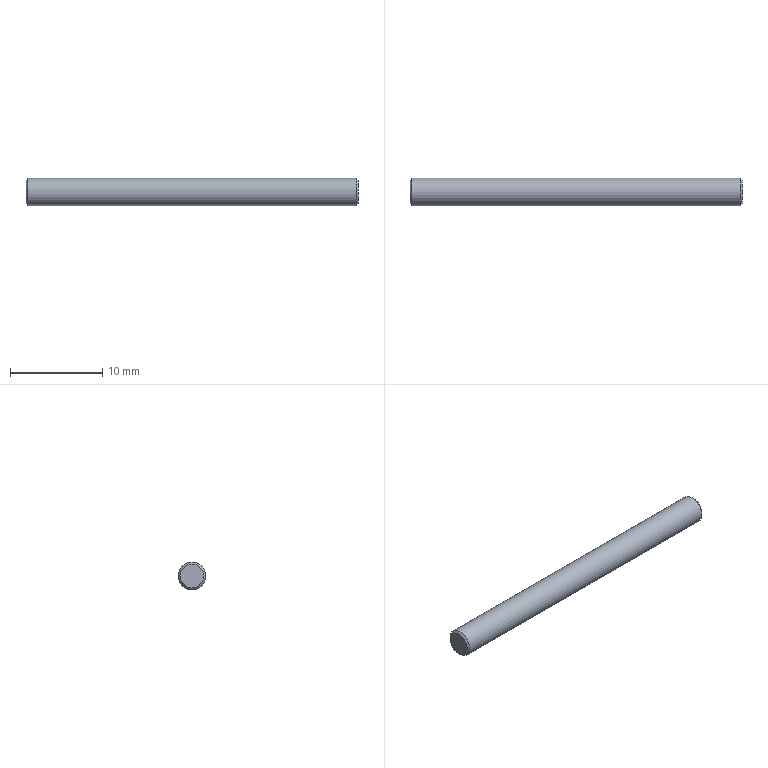Component | NX | SUPPORT_PIN | 1 solid | 5 faces | box 36 x 3 x 3 mm | volume 254 mm3 | plane 2 | cone 2 | cylinder 1 | commonest cylinder face diameters 3 x1
STEP:
#1=CARTESIAN_POINT('',(0.,0.,0.));
#2=DIRECTION('',(0.,0.,1.));
#3=DIRECTION('',(1.,0.,0.));
#4=AXIS2_PLACEMENT_3D('',#1,#2,#3);
#5=CARTESIAN_POINT('',(12.295,120.395,139.614));
#6=VERTEX_POINT('',#5);
#7=CARTESIAN_POINT('',(12.295,120.395,138.114));
#8=DIRECTION('',(-1.,0.,0.));
#9=DIRECTION('',(0.,0.,1.));
#10=AXIS2_PLACEMENT_3D('',#7,#8,#9);
#11=CIRCLE('',#10,1.5);
#12=CARTESIAN_POINT('',(-23.505,120.395,138.114));
#13=DIRECTION('',(1.,0.,0.));
#14=DIRECTION('',(0.,0.,-1.));
#15=AXIS2_PLACEMENT_3D('',#12,#13,#14);
#16=CYLINDRICAL_SURFACE('',#15,1.5);
#17=CARTESIAN_POINT('',(9.425,35.8));
#18=DIRECTION('',(-1.,0.));
#19=VECTOR('',#18,1.);
#20=LINE('',#17,#19);
#21=(GEOMETRIC_REPRESENTATION_CONTEXT(2)PARAMETRIC_REPRESENTATION_CONTEXT()REPRESENTATION_CONTEXT('',''));
#22=DEFINITIONAL_REPRESENTATION('',(#20),#21);
#23=PCURVE('',#16,#22);
#24=CARTESIAN_POINT('',(12.295,120.395,138.114));
#25=DIRECTION('',(-1.,0.,0.));
#26=DIRECTION('',(0.,0.,1.));
#27=AXIS2_PLACEMENT_3D('',#24,#25,#26);
#28=CONICAL_SURFACE('',#27,1.5,0.7854);
#29=CARTESIAN_POINT('',(0.,0.));
#30=DIRECTION('',(1.,0.));
#31=VECTOR('',#30,1.);
#32=LINE('',#29,#31);
#33=(GEOMETRIC_REPRESENTATION_CONTEXT(2)PARAMETRIC_REPRESENTATION_CONTEXT()REPRESENTATION_CONTEXT('',''));
#34=DEFINITIONAL_REPRESENTATION('',(#32),#33);
#35=PCURVE('',#28,#34);
#36=SURFACE_CURVE('',#11,(#23,#35),.PCURVE_S1.);
#37=EDGE_CURVE('',#6,#6,#36,.T.);
#38=ORIENTED_EDGE('',*,*,#37,.T.);
#39=CARTESIAN_POINT('',(-23.305,120.395,139.614));
#40=VERTEX_POINT('',#39);
#41=CARTESIAN_POINT('',(-23.305,120.395,139.614));
#42=CARTESIAN_POINT('',(12.295,120.395,139.614));
#43=B_SPLINE_CURVE_WITH_KNOTS('',1,(#41,#42),.UNSPECIFIED.,.F.,.F.,(2,2),(0.2,35.8),.PIECEWISE_BEZIER_KNOTS.);
#44=CARTESIAN_POINT('',(3.142,0.));
#45=DIRECTION('',(0.,1.));
#46=VECTOR('',#45,1.);
#47=LINE('',#44,#46);
#48=(GEOMETRIC_REPRESENTATION_CONTEXT(2)PARAMETRIC_REPRESENTATION_CONTEXT()REPRESENTATION_CONTEXT('',''));
#49=DEFINITIONAL_REPRESENTATION('',(#47),#48);
#50=PCURVE('',#16,#49);
#51=CARTESIAN_POINT('',(9.425,0.));
#52=DIRECTION('',(0.,1.));
#53=VECTOR('',#52,1.);
#54=LINE('',#51,#53);
#55=(GEOMETRIC_REPRESENTATION_CONTEXT(2)PARAMETRIC_REPRESENTATION_CONTEXT()REPRESENTATION_CONTEXT('',''));
#56=DEFINITIONAL_REPRESENTATION('',(#54),#55);
#57=PCURVE('',#16,#56);
#58=SEAM_CURVE('',#43,(#50,#57),.PCURVE_S1.);
#59=EDGE_CURVE('',#40,#6,#58,.T.);
#60=ORIENTED_EDGE('',*,*,#59,.F.);
#61=CARTESIAN_POINT('',(-23.305,120.395,138.114));
#62=DIRECTION('',(1.,0.,0.));
#63=DIRECTION('',(0.,0.,1.));
#64=AXIS2_PLACEMENT_3D('',#61,#62,#63);
#65=CIRCLE('',#64,1.5);
#66=CARTESIAN_POINT('',(3.142,0.2));
#67=DIRECTION('',(1.,0.));
#68=VECTOR('',#67,1.);
#69=LINE('',#66,#68);
#70=(GEOMETRIC_REPRESENTATION_CONTEXT(2)PARAMETRIC_REPRESENTATION_CONTEXT()REPRESENTATION_CONTEXT('',''));
#71=DEFINITIONAL_REPRESENTATION('',(#69),#70);
#72=PCURVE('',#16,#71);
#73=CARTESIAN_POINT('',(-23.505,120.395,138.114));
#74=DIRECTION('',(1.,0.,0.));
#75=DIRECTION('',(0.,0.,-1.));
#76=AXIS2_PLACEMENT_3D('',#73,#74,#75);
#77=CONICAL_SURFACE('',#76,1.3,0.7854);
#78=CARTESIAN_POINT('',(3.142,0.2));
#79=DIRECTION('',(1.,0.));
#80=VECTOR('',#79,1.);
#81=LINE('',#78,#80);
#82=(GEOMETRIC_REPRESENTATION_CONTEXT(2)PARAMETRIC_REPRESENTATION_CONTEXT()REPRESENTATION_CONTEXT('',''));
#83=DEFINITIONAL_REPRESENTATION('',(#81),#82);
#84=PCURVE('',#77,#83);
#85=SURFACE_CURVE('',#65,(#72,#84),.PCURVE_S1.);
#86=EDGE_CURVE('',#40,#40,#85,.T.);
#87=ORIENTED_EDGE('',*,*,#86,.T.);
#88=ORIENTED_EDGE('',*,*,#59,.T.);
#89=EDGE_LOOP('',(#38,#60,#87,#88));
#90=FACE_BOUND('',#89,.T.);
#91=ADVANCED_FACE('',(#90),#16,.T.);
#92=CARTESIAN_POINT('',(-23.505,120.395,139.414));
#93=VERTEX_POINT('',#92);
#94=CARTESIAN_POINT('',(-23.505,120.395,138.114));
#95=DIRECTION('',(-1.,0.,0.));
#96=DIRECTION('',(0.,0.,1.));
#97=AXIS2_PLACEMENT_3D('',#94,#95,#96);
#98=CIRCLE('',#97,1.3);
#99=CARTESIAN_POINT('',(-23.505,120.395,138.114));
#100=DIRECTION('',(-1.,0.,0.));
#101=DIRECTION('',(0.,0.,1.));
#102=AXIS2_PLACEMENT_3D('',#99,#100,#101);
#103=PLANE('',#102);
#104=CARTESIAN_POINT('',(0.,0.));
#105=DIRECTION('',(1.,0.));
#106=AXIS2_PLACEMENT_2D('',#104,#105);
#107=CIRCLE('',#106,1.3);
#108=(GEOMETRIC_REPRESENTATION_CONTEXT(2)PARAMETRIC_REPRESENTATION_CONTEXT()REPRESENTATION_CONTEXT('',''));
#109=DEFINITIONAL_REPRESENTATION('',(#107),#108);
#110=PCURVE('',#103,#109);
#111=CARTESIAN_POINT('',(9.425,0.));
#112=DIRECTION('',(-1.,0.));
#113=VECTOR('',#112,1.);
#114=LINE('',#111,#113);
#115=(GEOMETRIC_REPRESENTATION_CONTEXT(2)PARAMETRIC_REPRESENTATION_CONTEXT()REPRESENTATION_CONTEXT('',''));
#116=DEFINITIONAL_REPRESENTATION('',(#114),#115);
#117=PCURVE('',#77,#116);
#118=SURFACE_CURVE('',#98,(#110,#117),.PCURVE_S1.);
#119=EDGE_CURVE('',#93,#93,#118,.T.);
#120=ORIENTED_EDGE('',*,*,#119,.T.);
#121=EDGE_LOOP('',(#120));
#122=FACE_BOUND('',#121,.T.);
#123=ADVANCED_FACE('',(#122),#103,.T.);
#124=CARTESIAN_POINT('',(12.495,120.395,139.414));
#125=VERTEX_POINT('',#124);
#126=CARTESIAN_POINT('',(12.495,120.395,138.114));
#127=DIRECTION('',(1.,0.,0.));
#128=DIRECTION('',(0.,0.,1.));
#129=AXIS2_PLACEMENT_3D('',#126,#127,#128);
#130=CIRCLE('',#129,1.3);
#131=CARTESIAN_POINT('',(12.495,120.395,138.114));
#132=DIRECTION('',(-1.,0.,0.));
#133=DIRECTION('',(0.,0.,1.));
#134=AXIS2_PLACEMENT_3D('',#131,#132,#133);
#135=PLANE('',#134);
#136=CARTESIAN_POINT('',(1.3,0.));
#137=CARTESIAN_POINT('',(1.3,-2.252));
#138=CARTESIAN_POINT('',(-0.65,-1.126));
#139=CARTESIAN_POINT('',(-2.6,-0.));
#140=CARTESIAN_POINT('',(-0.65,1.126));
#141=CARTESIAN_POINT('',(1.3,2.252));
#142=CARTESIAN_POINT('',(1.3,0.));
#143=(BOUNDED_CURVE()B_SPLINE_CURVE(2,(#136,#137,#138,#139,#140,#141,#142),.UNSPECIFIED.,.T.,.F.)B_SPLINE_CURVE_WITH_KNOTS((1,2,2,2,2,1),(-2.094,0.,2.094,4.189,6.283,8.378),.UNSPECIFIED.)CURVE()GEOMETRIC_REPRESENTATION_ITEM()RATIONAL_B_SPLINE_CURVE((1.,0.5,1.,0.5,1.,0.5,1.))REPRESENTATION_ITEM(''));
#144=(GEOMETRIC_REPRESENTATION_CONTEXT(2)PARAMETRIC_REPRESENTATION_CONTEXT()REPRESENTATION_CONTEXT('',''));
#145=DEFINITIONAL_REPRESENTATION('',(#143),#144);
#146=PCURVE('',#135,#145);
#147=CARTESIAN_POINT('',(6.283,-0.2));
#148=DIRECTION('',(-1.,0.));
#149=VECTOR('',#148,1.);
#150=LINE('',#147,#149);
#151=(GEOMETRIC_REPRESENTATION_CONTEXT(2)PARAMETRIC_REPRESENTATION_CONTEXT()REPRESENTATION_CONTEXT('',''));
#152=DEFINITIONAL_REPRESENTATION('',(#150),#151);
#153=PCURVE('',#28,#152);
#154=SURFACE_CURVE('',#130,(#146,#153),.PCURVE_S1.);
#155=EDGE_CURVE('',#125,#125,#154,.T.);
#156=ORIENTED_EDGE('',*,*,#155,.T.);
#157=EDGE_LOOP('',(#156));
#158=FACE_BOUND('',#157,.T.);
#159=ADVANCED_FACE('',(#158),#135,.F.);
#160=ORIENTED_EDGE('',*,*,#155,.F.);
#161=CARTESIAN_POINT('',(12.495,120.395,139.414));
#162=CARTESIAN_POINT('',(12.295,120.395,139.614));
#163=B_SPLINE_CURVE_WITH_KNOTS('',1,(#161,#162),.UNSPECIFIED.,.F.,.F.,(2,2),(-0.2828,0.),.PIECEWISE_BEZIER_KNOTS.);
#164=CARTESIAN_POINT('',(6.283,0.));
#165=DIRECTION('',(0.,1.));
#166=VECTOR('',#165,1.);
#167=LINE('',#164,#166);
#168=(GEOMETRIC_REPRESENTATION_CONTEXT(2)PARAMETRIC_REPRESENTATION_CONTEXT()REPRESENTATION_CONTEXT('',''));
#169=DEFINITIONAL_REPRESENTATION('',(#167),#168);
#170=PCURVE('',#28,#169);
#171=CARTESIAN_POINT('',(0.,0.));
#172=DIRECTION('',(0.,1.));
#173=VECTOR('',#172,1.);
#174=LINE('',#171,#173);
#175=(GEOMETRIC_REPRESENTATION_CONTEXT(2)PARAMETRIC_REPRESENTATION_CONTEXT()REPRESENTATION_CONTEXT('',''));
#176=DEFINITIONAL_REPRESENTATION('',(#174),#175);
#177=PCURVE('',#28,#176);
#178=SEAM_CURVE('',#163,(#170,#177),.PCURVE_S1.);
#179=EDGE_CURVE('',#125,#6,#178,.T.);
#180=ORIENTED_EDGE('',*,*,#179,.T.);
#181=ORIENTED_EDGE('',*,*,#37,.F.);
#182=ORIENTED_EDGE('',*,*,#179,.F.);
#183=EDGE_LOOP('',(#160,#180,#181,#182));
#184=FACE_BOUND('',#183,.T.);
#185=ADVANCED_FACE('',(#184),#28,.T.);
#186=ORIENTED_EDGE('',*,*,#86,.F.);
#187=CARTESIAN_POINT('',(-23.505,120.395,139.414));
#188=CARTESIAN_POINT('',(-23.305,120.395,139.614));
#189=B_SPLINE_CURVE_WITH_KNOTS('',1,(#187,#188),.UNSPECIFIED.,.F.,.F.,(2,2),(0.,0.2828),.PIECEWISE_BEZIER_KNOTS.);
#190=CARTESIAN_POINT('',(3.142,0.));
#191=DIRECTION('',(0.,1.));
#192=VECTOR('',#191,1.);
#193=LINE('',#190,#192);
#194=(GEOMETRIC_REPRESENTATION_CONTEXT(2)PARAMETRIC_REPRESENTATION_CONTEXT()REPRESENTATION_CONTEXT('',''));
#195=DEFINITIONAL_REPRESENTATION('',(#193),#194);
#196=PCURVE('',#77,#195);
#197=CARTESIAN_POINT('',(9.425,0.));
#198=DIRECTION('',(0.,1.));
#199=VECTOR('',#198,1.);
#200=LINE('',#197,#199);
#201=(GEOMETRIC_REPRESENTATION_CONTEXT(2)PARAMETRIC_REPRESENTATION_CONTEXT()REPRESENTATION_CONTEXT('',''));
#202=DEFINITIONAL_REPRESENTATION('',(#200),#201);
#203=PCURVE('',#77,#202);
#204=SEAM_CURVE('',#189,(#196,#203),.PCURVE_S1.);
#205=EDGE_CURVE('',#93,#40,#204,.T.);
#206=ORIENTED_EDGE('',*,*,#205,.F.);
#207=ORIENTED_EDGE('',*,*,#119,.F.);
#208=ORIENTED_EDGE('',*,*,#205,.T.);
#209=EDGE_LOOP('',(#186,#206,#207,#208));
#210=FACE_BOUND('',#209,.T.);
#211=ADVANCED_FACE('',(#210),#77,.T.);
#212=CLOSED_SHELL('',(#91,#123,#159,#185,#211));
#213=MANIFOLD_SOLID_BREP('',#212);
#214=(LENGTH_UNIT()NAMED_UNIT(*)SI_UNIT(.MILLI.,.METRE.));
#215=UNCERTAINTY_MEASURE_WITH_UNIT(LENGTH_MEASURE(0.00001),#214,'','');
#216=(NAMED_UNIT(*)PLANE_ANGLE_UNIT()SI_UNIT($,.RADIAN.));
#217=(NAMED_UNIT(*)SI_UNIT($,.STERADIAN.)SOLID_ANGLE_UNIT());
#218=(GEOMETRIC_REPRESENTATION_CONTEXT(3)GLOBAL_UNCERTAINTY_ASSIGNED_CONTEXT((#215))GLOBAL_UNIT_ASSIGNED_CONTEXT((#214,#216,#217))REPRESENTATION_CONTEXT('',''));
#219=ADVANCED_BREP_SHAPE_REPRESENTATION('',(#4,#213),#218);